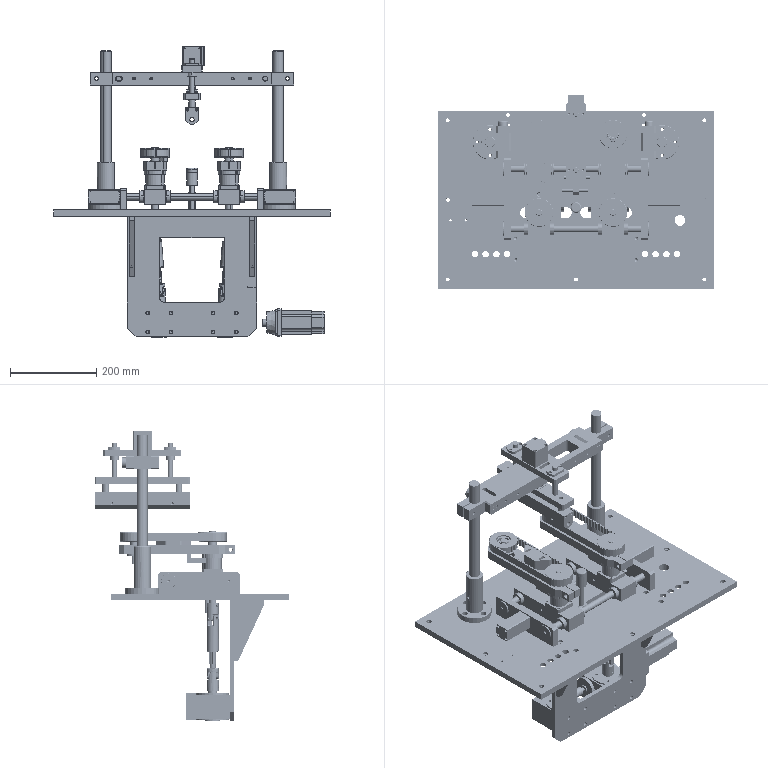Assembly | SolidWorks | mm | 92 component files | 92 solids | 4357 faces | box 643 x 451.5 x 676 mm | volume 10242694 mm3 | cylinder 1801 | plane 1479 | cone 493 | torus 376 | sphere 192 | spline 16 | commonest cylinder face diameters 5 x144 15 x118 6.5 x102 56 x84 62 x80 4 x76 9 x58 13 x56
Bill of materials:
CylinderFixingPlate | 1 |  | Rectangular flat plate with chamfered corners and a symmetric pattern of holes: three large round holes along the centerline, two elongated slots, four medium round holes around the central large hole, and four small holes beside the two end holes.
Fastener | 1 |  | Formed hat-profile strip bracket: a raised flat center section joined by two bends to two lower flanges. The center section has a U-shaped open slot coming in from one edge, and each flange has one round hole.
FlangeSeat | 2 |  | Flanged tubular boss: a round flange with four equally spaced holes and a hollow cylindrical tube standing up from it. The tube has a central bore and one small radial cross hole in its wall.
GuidePost | 2 |  | Stepped solid cylindrical pin: a long main diameter that steps down to a shorter, smaller-diameter end section.
LMH12UULinearBearing | 2 |  | Flanged cylindrical bushing-type part: a cylindrical body with a thicker flange at one end. The flange is round with two parallel flats, and it has a large central bore plus two smaller holes, one on each side.
MainArm | 1 |  | Elongated rectangular bar with forked (open-slotted) ends. It has two rectangular windows in the middle and small holes on the top and side faces, including through holes across the fork arms.
Pin | 1 |  | Headed cylindrical pin: a plain round shank with a larger, short cylindrical head at one end.
PinShaft | 1 |  | Headed cylindrical pin very similar to unnamed part. It has a plain round shank and a larger cylindrical head, and the head edge is visibly chamfered.
SDA32X20 | 1 |  | Roughly cubic block with chamfered vertical corners and four corner through holes. A rectangular tab sticks out from one side and has two holes in it, and a stepped round boss projects from the bottom.
ThermalInsulationSleeve | 2 |  | Plain cylindrical tube or spacer with a concentric through bore.
ThrustStud | 1 |  | Stepped solid shaft. Two cylindrical diameters lead to a larger collar that has at least one flat. Below the collar are a narrow groove (neck) and an end flange.
TransitionPlate | 1 |  | Rectangular flat bar with chamfered corners and holes along the centerline: a large hole near each end, a medium hole inboard of each, and two small holes near the center.
VerticalSealGuideAxis | 2 |  | Plain solid cylindrical rod with flat ends; long and slender.
VerticalSealMainArmFixingFrame | 2 |  | Rectangular block with a large through bore. A narrow slit runs from the bore to one end face, splitting that end. Two through holes cross the block side to side, and the two vertical edges at the opposite end are chamfered.
VerticalSealRoller | 1 |  | Long prismatic bar with a five-sided end profile: a rectangle whose lower corners are cut at an angle. A larger hole runs the length of the bar, two blind holes with cone-shaped bottoms sit in the end face, and two small holes are on the top face near the ends.
400WMotor | 1 |  | Body with a square flange: a flange plate with rounded corners and four corner holes, a short round pilot boss and a smaller cylindrical shaft sticking out from one face. Behind the flange is a long, nearly square body with concave rounded channels along its corners. The body steps to a slightly smaller section partway along, with a thin dividing line or groove at the step.
AdjustmentNut | 1 |  | Short plain cylindrical sleeve or tube with a concentric through bore and flat ends.
AdjustmentRod | 1 |  | Slender solid cylindrical rod or pin with small chamfers at both ends.
AxisEndCap | 6 |  | Thin flat circular disc with a small concentric through hole, like a washer. One face appears to have a small edge chamfer on the outer edge.
AxisSleeve | 2 |  | Tubular body with a through bore and a square mounting flange partway along its length. The flange has chamfered corners and four holes. Above the flange is a raised round collar with small side notches or flats, and the upper bore shows an internal step or groove near the top.
BearingLM16LUU | 4 |  | Cylindrical tube or sleeve with a concentric through bore and two narrow shallow grooves around the outside, one near each end.
Connector | 1 |  | Flange adapter: a square plate with chamfered corners, four small corner holes and a large central circular opening, with a short tapered, roughly conical tubular collar on one side. The iso view shows an irregular curved cut edge inside the collar.
CrossJoint | 4 |  | Short solid cylinder with well-rounded end edges. It has a centered axial hole, and a flat machined on one side with a radial hole through it.
DeepGrooveBallBearing6003_DeepGrooveBallBearing6003 | 4 |  | The geometry looks like a radial ball bearing: concentric outer and inner rings with a single row of balls between them (about 17 counted). No cage or shields are visible.
DeepGrooveBallBearing6202_DeepGrooveBallBearing6202 | 2 |  | Annular ring assembly-like solid: an outer ring and an inner ring, concentric, with a circle of spherical elements between them; resembles an open (unshielded) ball bearing.
DrivenWheel | 2 |  | Toothed cylindrical pulley-like part with a thin flange at each end and a stepped central through bore.
DriveWheel | 2 |  | Toothed cylindrical pulley-like part with a flange at each end and a keyed central through bore.
DriveWheelDriveAxis | 2 |  | Long slender stepped shaft with a raised collar near one end and reduced-diameter end journals with flat or keyway slot features.
FilmPullingFixingBase | 1 |  | Flat rectangular plate with a large rounded-corner rectangular window, two chamfered lower corners, and a pattern of through holes.
FilmPullingFixingBaseSupportPlate | 2 |  | Tapered gusset/bracket bar: a flat bar with a trapezoidal side profile and two countersunk or counterbored holes in its narrow top face.
FlangeClamp | 2 |  | L-shaped block: a base slab with a raised rear step, one vertical through hole, and a concave cylindrical cutout on the front end.
GearboxAxis | 2 |  | Short cylindrical pin/stub shaft with a raised collar near one end and elongated slot or flat features on both sides of the collar.
GuidePlate | 2 |  | Rectangular block with a large vertical through bore surrounded by four small holes, two large horizontal through bores near the ends, and a small cross hole in the side face.
GuideRod | 2 |  | Long, slender round rod with a small central hole or conical recess at the ends.
LimitAdjustmentScrew | 2 |  | Plain solid cylindrical rod with flat ends.
LongitudinalSealingPanel | 1 |  | Thin flat rectangular plate with two collinear slotted cutouts in the center and many through holes arranged in symmetric groups.
PositioningScrewPlate | 1 |  | Rectangular block with two chamfered top corners and two through holes near the top edge of the large face.
RubberPad | 1 |  | Solid stepped cylinder: a larger-diameter head with a rounded top edge above a smaller-diameter cylindrical shank, similar in form to a plug or cap.
SDA20X55 | 2 |  | Elongated rectangular box body with chamfered longitudinal edges; one end face has four corner holes and a small stepped cylindrical boss projecting from it.
Spline | 2 |  | Long slender shaft with longitudinal splines or ribs, a central axial hole at one end, a slightly reduced-diameter section near the other end, and a small cross hole near that end.
SupportPlate | 2 |  | Flat rectangular bar plate with two chamfered top corners, two larger holes near the ends, and a central large hole surrounded by four smaller holes in a square pattern.
SynchronousBelt | 2 |  | Closed-loop band with an elongated (stadium-shaped) path and regularly spaced teeth on the inner surface, resembling a toothed belt.
SynchronousBeltPressureBlock | 1 |  | Thick plate with a trapezoidal/truncated-triangle outline and rounded corners, with two parallel elongated slots through its thickness.
TensionConnectionAxis | 2 |  | Turned stepped pin: a larger central collar section with a radial cross hole and a flat, a smaller upper end with a groove near the tip, and a smaller lower shank with a neck/groove.
TensionConnectionAxisPad | 1 |  | Flat annular washer-like disc with a central round hole and a chamfered outer edge on one side.
UniversalJointA | 4 |  | Hollow cylindrical sleeve whose lower end is cut into two flattened tabs with rounded ends (a fork/clevis-like form), with small cross holes in the tabs and holes in the upper tube wall.
UniversalJointB | 2 |  | Cylindrical ring hub with a keyed central bore, and two legs extending downward forming a U/fork shape, with a radial hole in the hub and round holes near the leg ends.
UniversalJointC | 2 |  | Cylindrical body with a splined internal bore at one end and a forked (two-prong) opposite end; each prong is flat with a rounded tip and a cross hole.
WheelTensionAdjustmentPlate | 2 |  | Long flat rectangular bar with a large through-bore near one end. A narrow saw-cut slit runs from that bore out to the end face, and a small cross hole passes through the split end. The bar narrows around the split end. The other end has chamfered corners and a long through-slot with rounded ends. Three small round holes sit along the bar between the slot and the bore. Geometrically this resembles a split-clamp arm.
WormGearReducerNRV30-10-L+R | 1 |  | Two matching box-shaped housings in a row, joined by a short shaft with a larger cylindrical section in the middle. On each housing, the top face has a raised circular boss with a central bore that has a keyway notch, plus four small holes around it. The side faces have small holes near the corners. Round flanges stick out from the housing sides along the shaft axis. On the far housing, the outer flange has a bolt-hole circle and a shaft end sticking out. Overall it resembles a pair of right-angle drive units joined by a shaft, but this is not confirmed.
Mates: